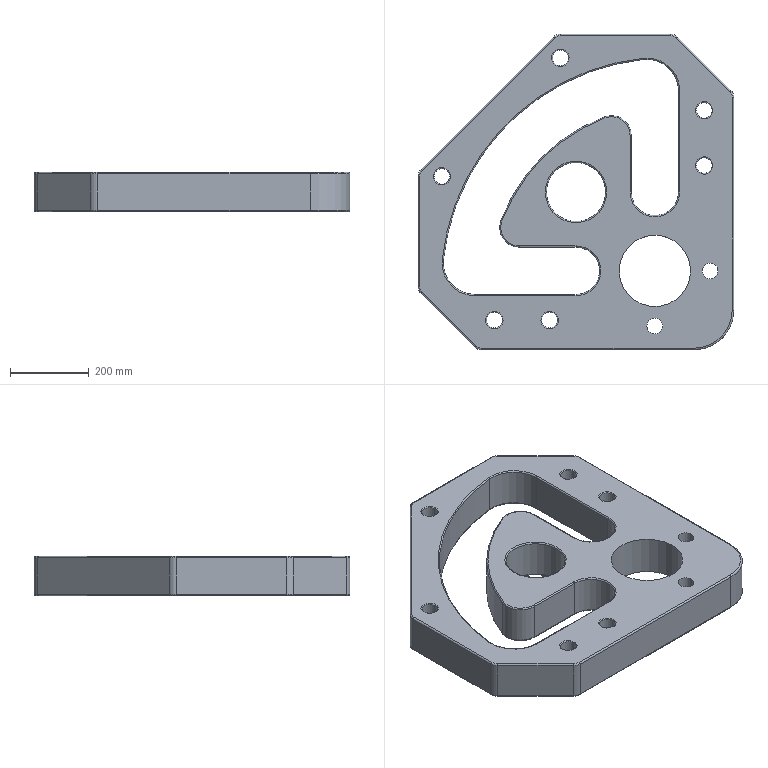Component | NX | A_PART_5 | 1 solid | 104 faces | volume 33468176 mm3 | cylinder 47 | torus 44 | plane 13 | commonest cylinder face diameters 8 x14 40 x8 6 x8 50 x6 160 x2 120 x2 100 x2 200 x1